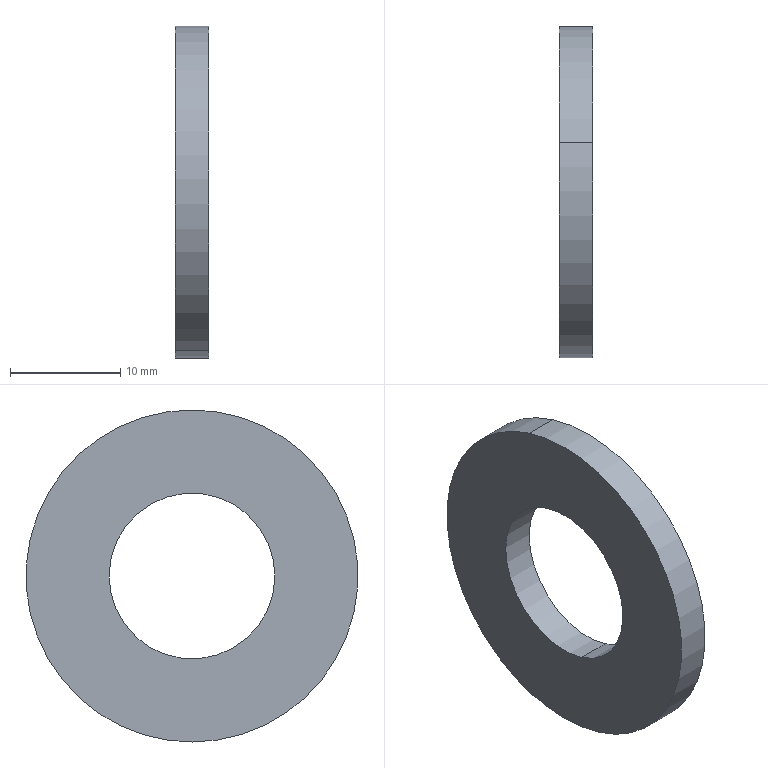Component | SolidWorks | ShaftRetainingRing-1 | 1 solid | 6 faces | box 3 x 30.05 x 30.05 mm | volume 1598 mm3 | cylinder 4 | plane 2 | commonest cylinder face diameters 15 x2 30.052 x2
build123d program:
from build123d import *

# Parameters (mm, degrees)
SKETCH2_R           = 15.026
SKETCH2_R_2         = 7.5
BOSS_EXTRUDE1_DEPTH = 3


with BuildPart() as part:
    # Sketch2 → Boss-Extrude1 (new body)
    with BuildSketch(Plane.XY):
        with Locations((0, 60.219)):
            Circle(SKETCH2_R)
        with Locations((0, 60.219)):
            Circle(SKETCH2_R_2, mode=Mode.SUBTRACT)
    extrude(amount=BOSS_EXTRUDE1_DEPTH)


solid = part.part

# Placed as in the assembly
solid = solid.moved(Location((-366, 0, 0), (0, 90, 0)))
STEP:
#1=COLOUR_RGB('',0.7922,0.8196,0.9333);
#2=FILL_AREA_STYLE_COLOUR('',#1);
#3=FILL_AREA_STYLE('',(#2));
#4=SURFACE_STYLE_FILL_AREA(#3);
#5=SURFACE_SIDE_STYLE('',(#4));
#6=SURFACE_STYLE_USAGE(.BOTH.,#5);
#7=PRESENTATION_STYLE_ASSIGNMENT((#6));
#8=CARTESIAN_POINT('',(-14.291,2.459,0.2819));
#9=VERTEX_POINT('',#8);
#10=CARTESIAN_POINT('',(-14.291,2.283,-0.2819));
#11=VERTEX_POINT('',#10);
#12=CARTESIAN_POINT('',(-14.291,2.371,0.));
#13=DIRECTION('',(1.,0.,-0.));
#14=DIRECTION('',(0.,-0.2971,-0.9548));
#15=AXIS2_PLACEMENT_3D('',#12,#13,#14);
#16=CIRCLE('',#15,0.2953);
#17=EDGE_CURVE('',#9,#11,#16,.T.);
#18=ORIENTED_EDGE('',*,*,#17,.T.);
#19=CARTESIAN_POINT('',(-14.409,2.283,-0.2819));
#20=VERTEX_POINT('',#19);
#21=CARTESIAN_POINT('',(-14.291,2.283,-0.2819));
#22=DIRECTION('',(-1.,-0.,0.));
#23=VECTOR('',#22,39.37);
#24=LINE('',#21,#23);
#25=EDGE_CURVE('',#11,#20,#24,.T.);
#26=ORIENTED_EDGE('',*,*,#25,.T.);
#27=CARTESIAN_POINT('',(-14.409,2.459,0.2819));
#28=VERTEX_POINT('',#27);
#29=CARTESIAN_POINT('',(-14.409,2.371,0.));
#30=DIRECTION('',(1.,0.,-0.));
#31=DIRECTION('',(0.,-0.2971,-0.9548));
#32=AXIS2_PLACEMENT_3D('',#29,#30,#31);
#33=CIRCLE('',#32,0.2953);
#34=EDGE_CURVE('',#28,#20,#33,.T.);
#35=ORIENTED_EDGE('',*,*,#34,.F.);
#36=CARTESIAN_POINT('',(-14.291,2.459,0.2819));
#37=DIRECTION('',(-1.,-0.,0.));
#38=VECTOR('',#37,39.37);
#39=LINE('',#36,#38);
#40=EDGE_CURVE('',#9,#28,#39,.T.);
#41=ORIENTED_EDGE('',*,*,#40,.F.);
#42=EDGE_LOOP('',(#18,#26,#35,#41));
#43=FACE_OUTER_BOUND('',#42,.T.);
#44=CARTESIAN_POINT('',(-14.291,2.371,0.));
#45=DIRECTION('',(-1.,-0.,0.));
#46=DIRECTION('',(0.,0.2971,0.9548));
#47=AXIS2_PLACEMENT_3D('',#44,#45,#46);
#48=CYLINDRICAL_SURFACE('',#47,0.2953);
#49=ADVANCED_FACE('',(#43),#48,.F.);
#50=CARTESIAN_POINT('',(-14.291,2.195,-0.5649));
#51=VERTEX_POINT('',#50);
#52=CARTESIAN_POINT('',(-14.291,2.547,0.5649));
#53=VERTEX_POINT('',#52);
#54=CARTESIAN_POINT('',(-14.291,2.371,0.));
#55=DIRECTION('',(1.,0.,-0.));
#56=DIRECTION('',(0.,-0.2971,-0.9548));
#57=AXIS2_PLACEMENT_3D('',#54,#55,#56);
#58=CIRCLE('',#57,0.5916);
#59=EDGE_CURVE('',#51,#53,#58,.T.);
#60=ORIENTED_EDGE('',*,*,#59,.F.);
#61=CARTESIAN_POINT('',(-14.409,2.195,-0.5649));
#62=VERTEX_POINT('',#61);
#63=CARTESIAN_POINT('',(-14.291,2.195,-0.5649));
#64=DIRECTION('',(-1.,-0.,0.));
#65=VECTOR('',#64,39.37);
#66=LINE('',#63,#65);
#67=EDGE_CURVE('',#51,#62,#66,.T.);
#68=ORIENTED_EDGE('',*,*,#67,.T.);
#69=CARTESIAN_POINT('',(-14.409,2.547,0.5649));
#70=VERTEX_POINT('',#69);
#71=CARTESIAN_POINT('',(-14.409,2.371,0.));
#72=DIRECTION('',(1.,0.,-0.));
#73=DIRECTION('',(0.,-0.2971,-0.9548));
#74=AXIS2_PLACEMENT_3D('',#71,#72,#73);
#75=CIRCLE('',#74,0.5916);
#76=EDGE_CURVE('',#62,#70,#75,.T.);
#77=ORIENTED_EDGE('',*,*,#76,.T.);
#78=CARTESIAN_POINT('',(-14.291,2.547,0.5649));
#79=DIRECTION('',(-1.,-0.,0.));
#80=VECTOR('',#79,39.37);
#81=LINE('',#78,#80);
#82=EDGE_CURVE('',#53,#70,#81,.T.);
#83=ORIENTED_EDGE('',*,*,#82,.F.);
#84=EDGE_LOOP('',(#60,#68,#77,#83));
#85=FACE_OUTER_BOUND('',#84,.T.);
#86=CARTESIAN_POINT('',(-14.291,2.371,0.));
#87=DIRECTION('',(-1.,-0.,0.));
#88=DIRECTION('',(0.,0.2971,0.9548));
#89=AXIS2_PLACEMENT_3D('',#86,#87,#88);
#90=CYLINDRICAL_SURFACE('',#89,0.5916);
#91=ADVANCED_FACE('',(#85),#90,.T.);
#92=CARTESIAN_POINT('',(-14.291,2.371,0.));
#93=DIRECTION('',(1.,0.,-0.));
#94=DIRECTION('',(0.,-0.2971,-0.9548));
#95=AXIS2_PLACEMENT_3D('',#92,#93,#94);
#96=CIRCLE('',#95,0.5916);
#97=EDGE_CURVE('',#53,#51,#96,.T.);
#98=ORIENTED_EDGE('',*,*,#97,.T.);
#99=ORIENTED_EDGE('',*,*,#59,.T.);
#100=EDGE_LOOP('',(#98,#99));
#101=FACE_OUTER_BOUND('',#100,.T.);
#102=ORIENTED_EDGE('',*,*,#17,.F.);
#103=CARTESIAN_POINT('',(-14.291,2.371,0.));
#104=DIRECTION('',(1.,0.,-0.));
#105=DIRECTION('',(0.,-0.2971,-0.9548));
#106=AXIS2_PLACEMENT_3D('',#103,#104,#105);
#107=CIRCLE('',#106,0.2953);
#108=EDGE_CURVE('',#11,#9,#107,.T.);
#109=ORIENTED_EDGE('',*,*,#108,.F.);
#110=EDGE_LOOP('',(#102,#109));
#111=FACE_BOUND('',#110,.T.);
#112=CARTESIAN_POINT('',(-14.291,2.371,0.));
#113=DIRECTION('',(1.,0.,-0.));
#114=DIRECTION('',(-0.,-0.2971,-0.9548));
#115=AXIS2_PLACEMENT_3D('',#112,#113,#114);
#116=PLANE('',#115);
#117=ADVANCED_FACE('',(#101,#111),#116,.T.);
#118=CARTESIAN_POINT('',(-14.409,2.371,0.));
#119=DIRECTION('',(1.,0.,-0.));
#120=DIRECTION('',(0.,-0.2971,-0.9548));
#121=AXIS2_PLACEMENT_3D('',#118,#119,#120);
#122=CIRCLE('',#121,0.5916);
#123=EDGE_CURVE('',#70,#62,#122,.T.);
#124=ORIENTED_EDGE('',*,*,#123,.F.);
#125=ORIENTED_EDGE('',*,*,#76,.F.);
#126=EDGE_LOOP('',(#124,#125));
#127=FACE_OUTER_BOUND('',#126,.T.);
#128=ORIENTED_EDGE('',*,*,#34,.T.);
#129=CARTESIAN_POINT('',(-14.409,2.371,0.));
#130=DIRECTION('',(1.,0.,-0.));
#131=DIRECTION('',(0.,-0.2971,-0.9548));
#132=AXIS2_PLACEMENT_3D('',#129,#130,#131);
#133=CIRCLE('',#132,0.2953);
#134=EDGE_CURVE('',#20,#28,#133,.T.);
#135=ORIENTED_EDGE('',*,*,#134,.T.);
#136=EDGE_LOOP('',(#128,#135));
#137=FACE_BOUND('',#136,.T.);
#138=CARTESIAN_POINT('',(-14.409,2.371,0.));
#139=DIRECTION('',(1.,0.,-0.));
#140=DIRECTION('',(-0.,-0.2971,-0.9548));
#141=AXIS2_PLACEMENT_3D('',#138,#139,#140);
#142=PLANE('',#141);
#143=ADVANCED_FACE('',(#127,#137),#142,.F.);
#144=ORIENTED_EDGE('',*,*,#67,.F.);
#145=ORIENTED_EDGE('',*,*,#97,.F.);
#146=ORIENTED_EDGE('',*,*,#82,.T.);
#147=ORIENTED_EDGE('',*,*,#123,.T.);
#148=EDGE_LOOP('',(#144,#145,#146,#147));
#149=FACE_OUTER_BOUND('',#148,.T.);
#150=CARTESIAN_POINT('',(-14.291,2.371,0.));
#151=DIRECTION('',(-1.,-0.,0.));
#152=DIRECTION('',(0.,0.2971,0.9548));
#153=AXIS2_PLACEMENT_3D('',#150,#151,#152);
#154=CYLINDRICAL_SURFACE('',#153,0.5916);
#155=ADVANCED_FACE('',(#149),#154,.T.);
#156=ORIENTED_EDGE('',*,*,#25,.F.);
#157=ORIENTED_EDGE('',*,*,#108,.T.);
#158=ORIENTED_EDGE('',*,*,#40,.T.);
#159=ORIENTED_EDGE('',*,*,#134,.F.);
#160=EDGE_LOOP('',(#156,#157,#158,#159));
#161=FACE_OUTER_BOUND('',#160,.T.);
#162=CARTESIAN_POINT('',(-14.291,2.371,0.));
#163=DIRECTION('',(-1.,-0.,0.));
#164=DIRECTION('',(0.,0.2971,0.9548));
#165=AXIS2_PLACEMENT_3D('',#162,#163,#164);
#166=CYLINDRICAL_SURFACE('',#165,0.2953);
#167=ADVANCED_FACE('',(#161),#166,.F.);
#168=CLOSED_SHELL('',(#49,#91,#117,#143,#155,#167));
#169=MANIFOLD_SOLID_BREP('',#168);
#170=STYLED_ITEM('',(#7),#169);
#171=(LENGTH_UNIT()NAMED_UNIT(*)SI_UNIT($,.METRE.));
#172=LENGTH_MEASURE_WITH_UNIT(LENGTH_MEASURE(0.0254),#171);
#173=DIMENSIONAL_EXPONENTS(1.,0.,0.,0.,0.,0.,0.);
#174=(CONVERSION_BASED_UNIT('',#172)LENGTH_UNIT()NAMED_UNIT(#173));
#175=UNCERTAINTY_MEASURE_WITH_UNIT(LENGTH_MEASURE(0.00001),#174,'','');
#176=(NAMED_UNIT(*)PLANE_ANGLE_UNIT()SI_UNIT($,.RADIAN.));
#177=(NAMED_UNIT(*)SI_UNIT($,.STERADIAN.)SOLID_ANGLE_UNIT());
#178=(GEOMETRIC_REPRESENTATION_CONTEXT(3)GLOBAL_UNCERTAINTY_ASSIGNED_CONTEXT((#175))GLOBAL_UNIT_ASSIGNED_CONTEXT((#174,#176,#177))REPRESENTATION_CONTEXT('',''));
#179=MECHANICAL_DESIGN_GEOMETRIC_PRESENTATION_REPRESENTATION('',(#170),#178);
#180=CARTESIAN_POINT('',(0.,0.,0.));
#181=DIRECTION('',(0.,0.,1.));
#182=DIRECTION('',(1.,0.,0.));
#183=AXIS2_PLACEMENT_3D('',#180,#181,#182);
#184=(LENGTH_UNIT()NAMED_UNIT(*)SI_UNIT($,.METRE.));
#185=LENGTH_MEASURE_WITH_UNIT(LENGTH_MEASURE(0.0254),#184);
#186=DIMENSIONAL_EXPONENTS(1.,0.,0.,0.,0.,0.,0.);
#187=(CONVERSION_BASED_UNIT('',#185)LENGTH_UNIT()NAMED_UNIT(#186));
#188=UNCERTAINTY_MEASURE_WITH_UNIT(LENGTH_MEASURE(0.00001),#187,'','');
#189=(NAMED_UNIT(*)PLANE_ANGLE_UNIT()SI_UNIT($,.RADIAN.));
#190=(NAMED_UNIT(*)SI_UNIT($,.STERADIAN.)SOLID_ANGLE_UNIT());
#191=(GEOMETRIC_REPRESENTATION_CONTEXT(3)GLOBAL_UNCERTAINTY_ASSIGNED_CONTEXT((#188))GLOBAL_UNIT_ASSIGNED_CONTEXT((#187,#189,#190))REPRESENTATION_CONTEXT('',''));
#192=ADVANCED_BREP_SHAPE_REPRESENTATION('',(#169,#183),#191);
#193=PRESENTATION_LAYER_ASSIGNMENT('','',(#170));